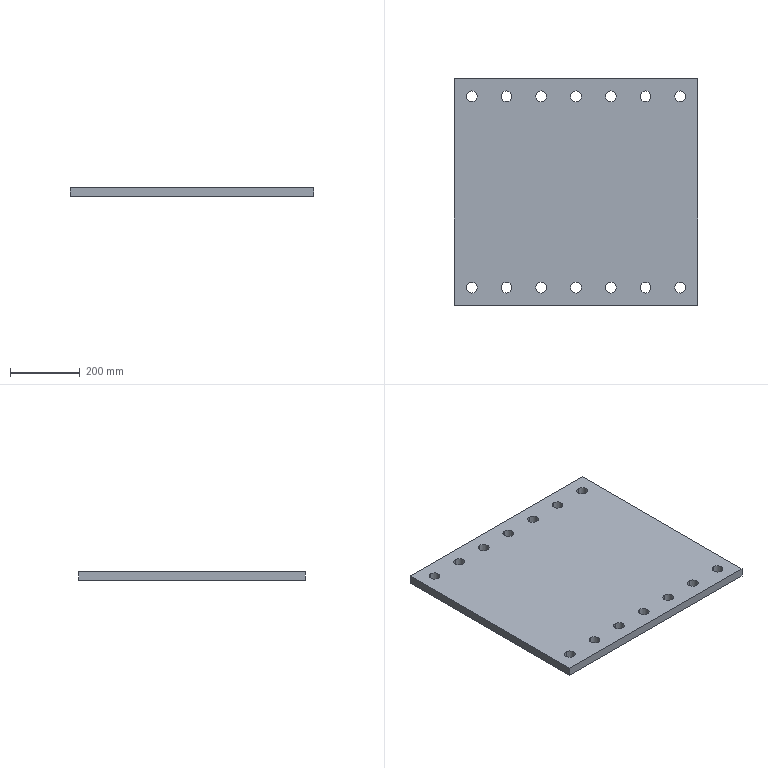Component | SolidWorks | 700X650X25-1 | 1 solid | 34 faces | volume 11110831 mm3 | cylinder 28 | plane 6 | commonest cylinder face diameters 31 x28 | material Plain Carbon Steel